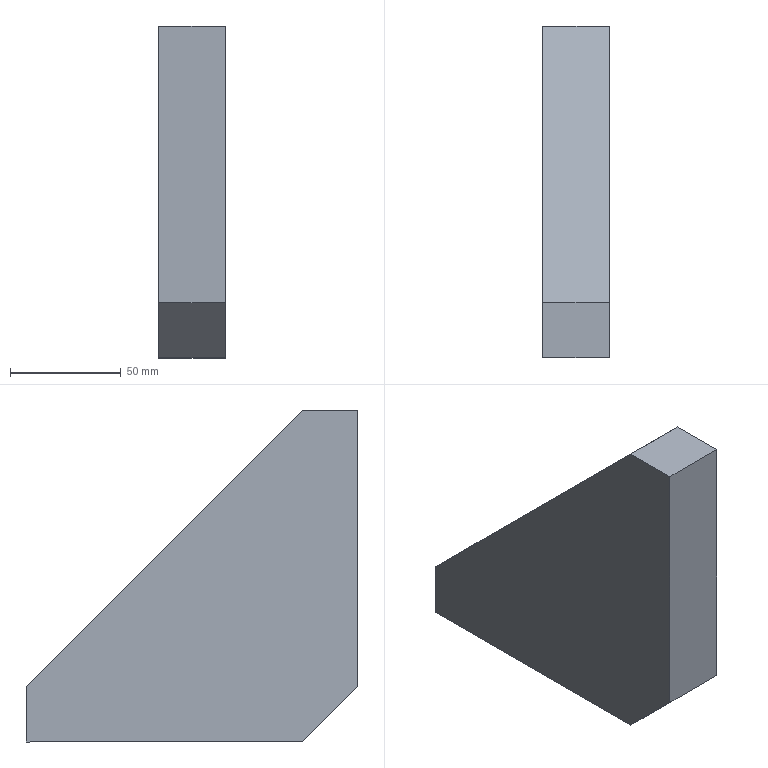Component | SolidWorks | BearingHousing-1_BearingHousingStiffener-1 | 1 solid | 8 faces | box 30 x 150 x 150 mm | volume 431250 mm3 | plane 8 | material Plain Carbon Steel
STEP:
#1=CARTESIAN_POINT('',(420.257,138.257,265.12));
#2=VERTEX_POINT('',#1);
#3=CARTESIAN_POINT('',(420.257,133.336,265.12));
#4=VERTEX_POINT('',#3);
#5=CARTESIAN_POINT('',(420.257,138.257,265.12));
#6=DIRECTION('',(0.,-1.,0.));
#7=VECTOR('',#6,39.37);
#8=LINE('',#5,#7);
#9=EDGE_CURVE('',#2,#4,#8,.T.);
#10=ORIENTED_EDGE('',*,*,#9,.F.);
#11=CARTESIAN_POINT('',(421.438,138.257,265.12));
#12=VERTEX_POINT('',#11);
#13=CARTESIAN_POINT('',(421.438,138.257,265.12));
#14=DIRECTION('',(-1.,-0.,0.));
#15=VECTOR('',#14,39.37);
#16=LINE('',#13,#15);
#17=EDGE_CURVE('',#12,#2,#16,.T.);
#18=ORIENTED_EDGE('',*,*,#17,.F.);
#19=CARTESIAN_POINT('',(421.438,133.336,265.12));
#20=VERTEX_POINT('',#19);
#21=CARTESIAN_POINT('',(421.438,138.257,265.12));
#22=DIRECTION('',(0.,-1.,0.));
#23=VECTOR('',#22,39.37);
#24=LINE('',#21,#23);
#25=EDGE_CURVE('',#12,#20,#24,.T.);
#26=ORIENTED_EDGE('',*,*,#25,.T.);
#27=CARTESIAN_POINT('',(421.438,133.336,265.12));
#28=DIRECTION('',(-1.,-0.,0.));
#29=VECTOR('',#28,39.37);
#30=LINE('',#27,#29);
#31=EDGE_CURVE('',#20,#4,#30,.T.);
#32=ORIENTED_EDGE('',*,*,#31,.T.);
#33=EDGE_LOOP('',(#10,#18,#26,#32));
#34=FACE_OUTER_BOUND('',#33,.T.);
#35=CARTESIAN_POINT('',(421.438,138.257,265.12));
#36=DIRECTION('',(0.,-0.,-1.));
#37=DIRECTION('',(0.,-1.,0.));
#38=AXIS2_PLACEMENT_3D('',#35,#36,#37);
#39=PLANE('',#38);
#40=ADVANCED_FACE('',(#34),#39,.T.);
#41=CARTESIAN_POINT('',(420.257,138.257,266.104));
#42=VERTEX_POINT('',#41);
#43=CARTESIAN_POINT('',(420.257,138.257,265.12));
#44=DIRECTION('',(0.,-0.,-1.));
#45=VECTOR('',#44,39.37);
#46=LINE('',#43,#45);
#47=EDGE_CURVE('',#42,#2,#46,.T.);
#48=ORIENTED_EDGE('',*,*,#47,.F.);
#49=CARTESIAN_POINT('',(421.438,138.257,266.104));
#50=VERTEX_POINT('',#49);
#51=CARTESIAN_POINT('',(421.438,138.257,266.104));
#52=DIRECTION('',(-1.,-0.,0.));
#53=VECTOR('',#52,39.37);
#54=LINE('',#51,#53);
#55=EDGE_CURVE('',#50,#42,#54,.T.);
#56=ORIENTED_EDGE('',*,*,#55,.F.);
#57=CARTESIAN_POINT('',(421.438,138.257,265.12));
#58=DIRECTION('',(0.,-0.,-1.));
#59=VECTOR('',#58,39.37);
#60=LINE('',#57,#59);
#61=EDGE_CURVE('',#50,#12,#60,.T.);
#62=ORIENTED_EDGE('',*,*,#61,.T.);
#63=ORIENTED_EDGE('',*,*,#17,.T.);
#64=EDGE_LOOP('',(#48,#56,#62,#63));
#65=FACE_OUTER_BOUND('',#64,.T.);
#66=CARTESIAN_POINT('',(421.438,138.257,265.12));
#67=DIRECTION('',(-0.,1.,-0.));
#68=DIRECTION('',(0.,-0.,-1.));
#69=AXIS2_PLACEMENT_3D('',#66,#67,#68);
#70=PLANE('',#69);
#71=ADVANCED_FACE('',(#65),#70,.T.);
#72=CARTESIAN_POINT('',(420.257,133.336,271.025));
#73=VERTEX_POINT('',#72);
#74=CARTESIAN_POINT('',(420.257,138.257,266.104));
#75=DIRECTION('',(-0.,0.7071,-0.7071));
#76=VECTOR('',#75,39.37);
#77=LINE('',#74,#76);
#78=EDGE_CURVE('',#73,#42,#77,.T.);
#79=ORIENTED_EDGE('',*,*,#78,.F.);
#80=CARTESIAN_POINT('',(421.438,133.336,271.025));
#81=VERTEX_POINT('',#80);
#82=CARTESIAN_POINT('',(421.438,133.336,271.025));
#83=DIRECTION('',(-1.,-0.,0.));
#84=VECTOR('',#83,39.37);
#85=LINE('',#82,#84);
#86=EDGE_CURVE('',#81,#73,#85,.T.);
#87=ORIENTED_EDGE('',*,*,#86,.F.);
#88=CARTESIAN_POINT('',(421.438,138.257,266.104));
#89=DIRECTION('',(-0.,0.7071,-0.7071));
#90=VECTOR('',#89,39.37);
#91=LINE('',#88,#90);
#92=EDGE_CURVE('',#81,#50,#91,.T.);
#93=ORIENTED_EDGE('',*,*,#92,.T.);
#94=ORIENTED_EDGE('',*,*,#55,.T.);
#95=EDGE_LOOP('',(#79,#87,#93,#94));
#96=FACE_OUTER_BOUND('',#95,.T.);
#97=CARTESIAN_POINT('',(421.438,138.257,266.104));
#98=DIRECTION('',(-0.,0.7071,0.7071));
#99=DIRECTION('',(-0.,0.7071,-0.7071));
#100=AXIS2_PLACEMENT_3D('',#97,#98,#99);
#101=PLANE('',#100);
#102=ADVANCED_FACE('',(#96),#101,.T.);
#103=CARTESIAN_POINT('',(420.257,132.352,271.025));
#104=VERTEX_POINT('',#103);
#105=CARTESIAN_POINT('',(420.257,133.336,271.025));
#106=DIRECTION('',(-0.,1.,-0.));
#107=VECTOR('',#106,39.37);
#108=LINE('',#105,#107);
#109=EDGE_CURVE('',#104,#73,#108,.T.);
#110=ORIENTED_EDGE('',*,*,#109,.F.);
#111=CARTESIAN_POINT('',(421.438,132.352,271.025));
#112=VERTEX_POINT('',#111);
#113=CARTESIAN_POINT('',(421.438,132.352,271.025));
#114=DIRECTION('',(-1.,-0.,0.));
#115=VECTOR('',#114,39.37);
#116=LINE('',#113,#115);
#117=EDGE_CURVE('',#112,#104,#116,.T.);
#118=ORIENTED_EDGE('',*,*,#117,.F.);
#119=CARTESIAN_POINT('',(421.438,133.336,271.025));
#120=DIRECTION('',(-0.,1.,-0.));
#121=VECTOR('',#120,39.37);
#122=LINE('',#119,#121);
#123=EDGE_CURVE('',#112,#81,#122,.T.);
#124=ORIENTED_EDGE('',*,*,#123,.T.);
#125=ORIENTED_EDGE('',*,*,#86,.T.);
#126=EDGE_LOOP('',(#110,#118,#124,#125));
#127=FACE_OUTER_BOUND('',#126,.T.);
#128=CARTESIAN_POINT('',(421.438,133.336,271.025));
#129=DIRECTION('',(-0.,0.,1.));
#130=DIRECTION('',(-0.,1.,-0.));
#131=AXIS2_PLACEMENT_3D('',#128,#129,#130);
#132=PLANE('',#131);
#133=ADVANCED_FACE('',(#127),#132,.T.);
#134=CARTESIAN_POINT('',(420.257,132.352,266.104));
#135=VERTEX_POINT('',#134);
#136=CARTESIAN_POINT('',(420.257,132.352,266.104));
#137=DIRECTION('',(-0.,0.,1.));
#138=VECTOR('',#137,39.37);
#139=LINE('',#136,#138);
#140=EDGE_CURVE('',#135,#104,#139,.T.);
#141=ORIENTED_EDGE('',*,*,#140,.F.);
#142=CARTESIAN_POINT('',(421.438,132.352,266.104));
#143=VERTEX_POINT('',#142);
#144=CARTESIAN_POINT('',(421.438,132.352,266.104));
#145=DIRECTION('',(-1.,-0.,0.));
#146=VECTOR('',#145,39.37);
#147=LINE('',#144,#146);
#148=EDGE_CURVE('',#143,#135,#147,.T.);
#149=ORIENTED_EDGE('',*,*,#148,.F.);
#150=CARTESIAN_POINT('',(421.438,132.352,266.104));
#151=DIRECTION('',(-0.,0.,1.));
#152=VECTOR('',#151,39.37);
#153=LINE('',#150,#152);
#154=EDGE_CURVE('',#143,#112,#153,.T.);
#155=ORIENTED_EDGE('',*,*,#154,.T.);
#156=ORIENTED_EDGE('',*,*,#117,.T.);
#157=EDGE_LOOP('',(#141,#149,#155,#156));
#158=FACE_OUTER_BOUND('',#157,.T.);
#159=CARTESIAN_POINT('',(421.438,132.352,266.104));
#160=DIRECTION('',(0.,-1.,0.));
#161=DIRECTION('',(-0.,0.,1.));
#162=AXIS2_PLACEMENT_3D('',#159,#160,#161);
#163=PLANE('',#162);
#164=ADVANCED_FACE('',(#158),#163,.T.);
#165=CARTESIAN_POINT('',(420.257,133.336,265.12));
#166=DIRECTION('',(0.,-0.7071,0.7071));
#167=VECTOR('',#166,39.37);
#168=LINE('',#165,#167);
#169=EDGE_CURVE('',#4,#135,#168,.T.);
#170=ORIENTED_EDGE('',*,*,#169,.F.);
#171=ORIENTED_EDGE('',*,*,#31,.F.);
#172=CARTESIAN_POINT('',(421.438,133.336,265.12));
#173=DIRECTION('',(0.,-0.7071,0.7071));
#174=VECTOR('',#173,39.37);
#175=LINE('',#172,#174);
#176=EDGE_CURVE('',#20,#143,#175,.T.);
#177=ORIENTED_EDGE('',*,*,#176,.T.);
#178=ORIENTED_EDGE('',*,*,#148,.T.);
#179=EDGE_LOOP('',(#170,#171,#177,#178));
#180=FACE_OUTER_BOUND('',#179,.T.);
#181=CARTESIAN_POINT('',(421.438,133.336,265.12));
#182=DIRECTION('',(0.,-0.7071,-0.7071));
#183=DIRECTION('',(0.,-0.7071,0.7071));
#184=AXIS2_PLACEMENT_3D('',#181,#182,#183);
#185=PLANE('',#184);
#186=ADVANCED_FACE('',(#180),#185,.T.);
#187=ORIENTED_EDGE('',*,*,#25,.F.);
#188=ORIENTED_EDGE('',*,*,#61,.F.);
#189=ORIENTED_EDGE('',*,*,#92,.F.);
#190=ORIENTED_EDGE('',*,*,#123,.F.);
#191=ORIENTED_EDGE('',*,*,#154,.F.);
#192=ORIENTED_EDGE('',*,*,#176,.F.);
#193=EDGE_LOOP('',(#187,#188,#189,#190,#191,#192));
#194=FACE_OUTER_BOUND('',#193,.T.);
#195=CARTESIAN_POINT('',(421.438,138.257,265.12));
#196=DIRECTION('',(-1.,-0.,-0.));
#197=DIRECTION('',(0.,-1.,0.));
#198=AXIS2_PLACEMENT_3D('',#195,#196,#197);
#199=PLANE('',#198);
#200=ADVANCED_FACE('',(#194),#199,.F.);
#201=ORIENTED_EDGE('',*,*,#9,.T.);
#202=ORIENTED_EDGE('',*,*,#169,.T.);
#203=ORIENTED_EDGE('',*,*,#140,.T.);
#204=ORIENTED_EDGE('',*,*,#109,.T.);
#205=ORIENTED_EDGE('',*,*,#78,.T.);
#206=ORIENTED_EDGE('',*,*,#47,.T.);
#207=EDGE_LOOP('',(#201,#202,#203,#204,#205,#206));
#208=FACE_OUTER_BOUND('',#207,.T.);
#209=CARTESIAN_POINT('',(420.257,138.257,265.12));
#210=DIRECTION('',(-1.,-0.,-0.));
#211=DIRECTION('',(0.,-1.,0.));
#212=AXIS2_PLACEMENT_3D('',#209,#210,#211);
#213=PLANE('',#212);
#214=ADVANCED_FACE('',(#208),#213,.T.);
#215=CLOSED_SHELL('',(#40,#71,#102,#133,#164,#186,#200,#214));
#216=MANIFOLD_SOLID_BREP('',#215);
#217=CARTESIAN_POINT('',(0.,0.,0.));
#218=DIRECTION('',(0.,0.,1.));
#219=DIRECTION('',(1.,0.,0.));
#220=AXIS2_PLACEMENT_3D('',#217,#218,#219);
#221=(LENGTH_UNIT()NAMED_UNIT(*)SI_UNIT($,.METRE.));
#222=LENGTH_MEASURE_WITH_UNIT(LENGTH_MEASURE(0.0254),#221);
#223=DIMENSIONAL_EXPONENTS(1.,0.,0.,0.,0.,0.,0.);
#224=(CONVERSION_BASED_UNIT('',#222)LENGTH_UNIT()NAMED_UNIT(#223));
#225=UNCERTAINTY_MEASURE_WITH_UNIT(LENGTH_MEASURE(0.00001),#224,'','');
#226=(NAMED_UNIT(*)PLANE_ANGLE_UNIT()SI_UNIT($,.RADIAN.));
#227=(NAMED_UNIT(*)SI_UNIT($,.STERADIAN.)SOLID_ANGLE_UNIT());
#228=(GEOMETRIC_REPRESENTATION_CONTEXT(3)GLOBAL_UNCERTAINTY_ASSIGNED_CONTEXT((#225))GLOBAL_UNIT_ASSIGNED_CONTEXT((#224,#226,#227))REPRESENTATION_CONTEXT('',''));
#229=ADVANCED_BREP_SHAPE_REPRESENTATION('',(#216,#220),#228);
#230=COLOUR_RGB('',0.7922,0.8196,0.9333);
#231=FILL_AREA_STYLE_COLOUR('',#230);
#232=FILL_AREA_STYLE('',(#231));
#233=SURFACE_STYLE_FILL_AREA(#232);
#234=SURFACE_SIDE_STYLE('',(#233));
#235=SURFACE_STYLE_USAGE(.BOTH.,#234);
#236=PRESENTATION_STYLE_ASSIGNMENT((#235));
#237=STYLED_ITEM('',(#236),#216);
#238=PRESENTATION_LAYER_ASSIGNMENT('','',(#237));
#239=(LENGTH_UNIT()NAMED_UNIT(*)SI_UNIT($,.METRE.));
#240=LENGTH_MEASURE_WITH_UNIT(LENGTH_MEASURE(0.0254),#239);
#241=DIMENSIONAL_EXPONENTS(1.,0.,0.,0.,0.,0.,0.);
#242=(CONVERSION_BASED_UNIT('',#240)LENGTH_UNIT()NAMED_UNIT(#241));
#243=UNCERTAINTY_MEASURE_WITH_UNIT(LENGTH_MEASURE(0.00001),#242,'','');
#244=(NAMED_UNIT(*)PLANE_ANGLE_UNIT()SI_UNIT($,.RADIAN.));
#245=(NAMED_UNIT(*)SI_UNIT($,.STERADIAN.)SOLID_ANGLE_UNIT());
#246=(GEOMETRIC_REPRESENTATION_CONTEXT(3)GLOBAL_UNCERTAINTY_ASSIGNED_CONTEXT((#243))GLOBAL_UNIT_ASSIGNED_CONTEXT((#242,#244,#245))REPRESENTATION_CONTEXT('',''));
#247=MECHANICAL_DESIGN_GEOMETRIC_PRESENTATION_REPRESENTATION('',(#237),#246);